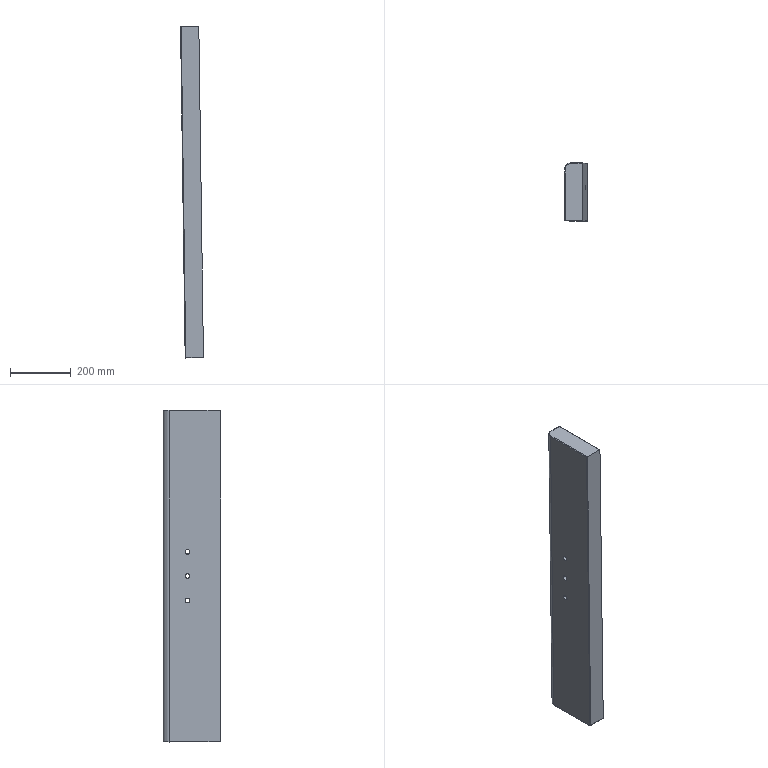Component | SolidWorks | DA-0220-Part8-5 | 1 solid | 23 faces | box 75.24 x 189.53 x 1090.68 mm | volume 12261983 mm3 | cylinder 14 | plane 6 | torus 2 | sphere 1 | commonest cylinder face diameters 4 x7 16 x6 40 x1
build123d program:
from build123d import *

# Parameters (mm, degrees)
SKETCH1_W           = 60
SKETCH1_H           = 189.5
BOSS_EXTRUDE1_DEPTH = 545
FILLET1_R           = 20
FILLET2_R           = 2
SKETCH1_2_R         = 8
CUT_EXTRUDE1_DEPTH  = 581.117


with BuildPart() as part:
    # Sketch1 → Boss-Extrude1 (new, symmetric)
    with BuildSketch(Plane.XY):
        with Locations((30, 94.75)):
            Rectangle(SKETCH1_W, SKETCH1_H)
    extrude(amount=BOSS_EXTRUDE1_DEPTH, both=True)

    # Fillet1
    fillet1_edges = [part.edges().sort_by_distance(p)[0] for p in [
        (60, 189.5, 0),
    ]]
    fillet(fillet1_edges, radius=FILLET1_R)

    # Fillet2
    fillet2_edges = [part.edges().sort_by_distance(p)[0] for p in [
        (20, 189.5, -545),
        (20, 189.5, 545),
        (54.142, 183.642, -545),
        (54.142, 183.642, 545),
        (30, 0, 545),
        (0, 94.75, -545),
        (60, 84.75, -545),
        (60, 84.75, 545),
        (60, 0, 0),
    ]]
    fillet(fillet2_edges, radius=FILLET2_R)

    # Sketch1_2 → Cut-Extrude1 (cut, through all)
    with BuildSketch(Plane(origin=(60, 0, 0), x_dir=(0, 0, -1), z_dir=(1, 0, 0))):
        with Locations(Location((80, 109.5, 0), (0, 0, 90))):
            Circle(SKETCH1_2_R)
        with Locations(Location((0, 109.5, 0), (0, 0, 90))):
            Circle(SKETCH1_2_R)
        with Locations(Location((-80, 109.5, 0), (0, 0, 90))):
            Circle(SKETCH1_2_R)
    extrude(amount=-CUT_EXTRUDE1_DEPTH, mode=Mode.SUBTRACT)


solid = part.part

# Placed as in the assembly
solid = solid.moved(Location((302.195, -203.43, 7.718), (-180, 0.7995, 179.977)))
STEP:
#1=CARTESIAN_POINT('',(11.94,-4.013,-2.845));
#2=VERTEX_POINT('',#1);
#3=CARTESIAN_POINT('',(11.94,-3.383,-2.845));
#4=VERTEX_POINT('',#3);
#5=CARTESIAN_POINT('',(11.94,-3.698,-2.845));
#6=DIRECTION('',(-0.9999,-0.000404,-0.01395));
#7=DIRECTION('',(-0.000404,1.,-0.00000282));
#8=AXIS2_PLACEMENT_3D('',#5,#6,#7);
#9=CIRCLE('',#8,0.315);
#10=EDGE_CURVE('',#2,#4,#9,.T.);
#11=ORIENTED_EDGE('',*,*,#10,.F.);
#12=CARTESIAN_POINT('',(9.578,-4.014,-2.878));
#13=VERTEX_POINT('',#12);
#14=CARTESIAN_POINT('',(11.94,-4.013,-2.845));
#15=DIRECTION('',(-0.9999,-0.000404,-0.01395));
#16=VECTOR('',#15,39.37);
#17=LINE('',#14,#16);
#18=EDGE_CURVE('',#2,#13,#17,.T.);
#19=ORIENTED_EDGE('',*,*,#18,.T.);
#20=CARTESIAN_POINT('',(9.578,-3.384,-2.878));
#21=VERTEX_POINT('',#20);
#22=CARTESIAN_POINT('',(9.578,-3.699,-2.878));
#23=DIRECTION('',(-0.9999,-0.000404,-0.01395));
#24=DIRECTION('',(-0.000404,1.,-0.00000282));
#25=AXIS2_PLACEMENT_3D('',#22,#23,#24);
#26=CIRCLE('',#25,0.315);
#27=EDGE_CURVE('',#13,#21,#26,.T.);
#28=ORIENTED_EDGE('',*,*,#27,.T.);
#29=CARTESIAN_POINT('',(11.94,-3.383,-2.845));
#30=DIRECTION('',(-0.9999,-0.000404,-0.01395));
#31=VECTOR('',#30,39.37);
#32=LINE('',#29,#31);
#33=EDGE_CURVE('',#4,#21,#32,.T.);
#34=ORIENTED_EDGE('',*,*,#33,.F.);
#35=EDGE_LOOP('',(#11,#19,#28,#34));
#36=FACE_OUTER_BOUND('',#35,.T.);
#37=CARTESIAN_POINT('',(11.94,-3.698,-2.845));
#38=DIRECTION('',(-0.9999,-0.000404,-0.01395));
#39=DIRECTION('',(-0.000404,1.,-0.00000282));
#40=AXIS2_PLACEMENT_3D('',#37,#38,#39);
#41=CYLINDRICAL_SURFACE('',#40,0.315);
#42=ADVANCED_FACE('',(#36),#41,.F.);
#43=CARTESIAN_POINT('',(11.896,-4.013,0.3038));
#44=VERTEX_POINT('',#43);
#45=CARTESIAN_POINT('',(11.896,-3.383,0.3038));
#46=VERTEX_POINT('',#45);
#47=CARTESIAN_POINT('',(11.896,-3.698,0.3038));
#48=DIRECTION('',(-0.9999,-0.000404,-0.01395));
#49=DIRECTION('',(-0.000404,1.,-0.00000282));
#50=AXIS2_PLACEMENT_3D('',#47,#48,#49);
#51=CIRCLE('',#50,0.315);
#52=EDGE_CURVE('',#44,#46,#51,.T.);
#53=ORIENTED_EDGE('',*,*,#52,.F.);
#54=CARTESIAN_POINT('',(9.534,-4.014,0.2709));
#55=VERTEX_POINT('',#54);
#56=CARTESIAN_POINT('',(11.896,-4.013,0.3038));
#57=DIRECTION('',(-0.9999,-0.000404,-0.01395));
#58=VECTOR('',#57,39.37);
#59=LINE('',#56,#58);
#60=EDGE_CURVE('',#44,#55,#59,.T.);
#61=ORIENTED_EDGE('',*,*,#60,.T.);
#62=CARTESIAN_POINT('',(9.534,-3.384,0.2709));
#63=VERTEX_POINT('',#62);
#64=CARTESIAN_POINT('',(9.534,-3.699,0.2709));
#65=DIRECTION('',(-0.9999,-0.000404,-0.01395));
#66=DIRECTION('',(-0.000404,1.,-0.00000282));
#67=AXIS2_PLACEMENT_3D('',#64,#65,#66);
#68=CIRCLE('',#67,0.315);
#69=EDGE_CURVE('',#55,#63,#68,.T.);
#70=ORIENTED_EDGE('',*,*,#69,.T.);
#71=CARTESIAN_POINT('',(11.896,-3.383,0.3038));
#72=DIRECTION('',(-0.9999,-0.000404,-0.01395));
#73=VECTOR('',#72,39.37);
#74=LINE('',#71,#73);
#75=EDGE_CURVE('',#46,#63,#74,.T.);
#76=ORIENTED_EDGE('',*,*,#75,.F.);
#77=EDGE_LOOP('',(#53,#61,#70,#76));
#78=FACE_OUTER_BOUND('',#77,.T.);
#79=CARTESIAN_POINT('',(11.896,-3.698,0.3038));
#80=DIRECTION('',(-0.9999,-0.000404,-0.01395));
#81=DIRECTION('',(-0.000404,1.,-0.00000282));
#82=AXIS2_PLACEMENT_3D('',#79,#80,#81);
#83=CYLINDRICAL_SURFACE('',#82,0.315);
#84=ADVANCED_FACE('',(#78),#83,.F.);
#85=CARTESIAN_POINT('',(11.852,-4.013,3.453));
#86=VERTEX_POINT('',#85);
#87=CARTESIAN_POINT('',(11.852,-3.383,3.453));
#88=VERTEX_POINT('',#87);
#89=CARTESIAN_POINT('',(11.852,-3.698,3.453));
#90=DIRECTION('',(-0.9999,-0.000404,-0.01395));
#91=DIRECTION('',(-0.000404,1.,-0.00000282));
#92=AXIS2_PLACEMENT_3D('',#89,#90,#91);
#93=CIRCLE('',#92,0.315);
#94=EDGE_CURVE('',#86,#88,#93,.T.);
#95=ORIENTED_EDGE('',*,*,#94,.F.);
#96=CARTESIAN_POINT('',(9.49,-4.014,3.42));
#97=VERTEX_POINT('',#96);
#98=CARTESIAN_POINT('',(11.852,-4.013,3.453));
#99=DIRECTION('',(-0.9999,-0.000404,-0.01395));
#100=VECTOR('',#99,39.37);
#101=LINE('',#98,#100);
#102=EDGE_CURVE('',#86,#97,#101,.T.);
#103=ORIENTED_EDGE('',*,*,#102,.T.);
#104=CARTESIAN_POINT('',(9.49,-3.384,3.42));
#105=VERTEX_POINT('',#104);
#106=CARTESIAN_POINT('',(9.49,-3.699,3.42));
#107=DIRECTION('',(-0.9999,-0.000404,-0.01395));
#108=DIRECTION('',(-0.000404,1.,-0.00000282));
#109=AXIS2_PLACEMENT_3D('',#106,#107,#108);
#110=CIRCLE('',#109,0.315);
#111=EDGE_CURVE('',#97,#105,#110,.T.);
#112=ORIENTED_EDGE('',*,*,#111,.T.);
#113=CARTESIAN_POINT('',(11.852,-3.383,3.453));
#114=DIRECTION('',(-0.9999,-0.000404,-0.01395));
#115=VECTOR('',#114,39.37);
#116=LINE('',#113,#115);
#117=EDGE_CURVE('',#88,#105,#116,.T.);
#118=ORIENTED_EDGE('',*,*,#117,.F.);
#119=EDGE_LOOP('',(#95,#103,#112,#118));
#120=FACE_OUTER_BOUND('',#119,.T.);
#121=CARTESIAN_POINT('',(11.852,-3.698,3.453));
#122=DIRECTION('',(-0.9999,-0.000404,-0.01395));
#123=DIRECTION('',(-0.000404,1.,-0.00000282));
#124=AXIS2_PLACEMENT_3D('',#121,#122,#123);
#125=CYLINDRICAL_SURFACE('',#124,0.315);
#126=ADVANCED_FACE('',(#120),#125,.F.);
#127=CARTESIAN_POINT('',(12.196,-8.009,-21.072));
#128=VERTEX_POINT('',#127);
#129=CARTESIAN_POINT('',(11.599,-8.009,21.68));
#130=VERTEX_POINT('',#129);
#131=CARTESIAN_POINT('',(12.197,-8.009,-21.151));
#132=DIRECTION('',(-0.01395,-0.00000282,0.9999));
#133=VECTOR('',#132,39.37);
#134=LINE('',#131,#133);
#135=EDGE_CURVE('',#128,#130,#134,.T.);
#136=ORIENTED_EDGE('',*,*,#135,.T.);
#137=CARTESIAN_POINT('',(11.519,-8.009,21.757));
#138=VERTEX_POINT('',#137);
#139=CARTESIAN_POINT('',(11.52,-8.009,21.679));
#140=DIRECTION('',(0.000404,-1.,0.00000282));
#141=DIRECTION('',(0.9999,0.000404,0.01395));
#142=AXIS2_PLACEMENT_3D('',#139,#140,#141);
#143=CIRCLE('',#142,0.07874);
#144=EDGE_CURVE('',#130,#138,#143,.T.);
#145=ORIENTED_EDGE('',*,*,#144,.T.);
#146=CARTESIAN_POINT('',(9.315,-8.01,21.727));
#147=VERTEX_POINT('',#146);
#148=CARTESIAN_POINT('',(9.236,-8.01,21.725));
#149=DIRECTION('',(-0.9999,-0.000404,-0.01395));
#150=VECTOR('',#149,39.37);
#151=LINE('',#148,#150);
#152=EDGE_CURVE('',#138,#147,#151,.T.);
#153=ORIENTED_EDGE('',*,*,#152,.T.);
#154=CARTESIAN_POINT('',(9.912,-8.01,-21.104));
#155=VERTEX_POINT('',#154);
#156=CARTESIAN_POINT('',(9.914,-8.01,-21.183));
#157=DIRECTION('',(0.01395,0.00000282,-0.9999));
#158=VECTOR('',#157,39.37);
#159=LINE('',#156,#158);
#160=EDGE_CURVE('',#147,#155,#159,.T.);
#161=ORIENTED_EDGE('',*,*,#160,.T.);
#162=CARTESIAN_POINT('',(9.834,-8.01,-21.105));
#163=DIRECTION('',(0.9999,0.000404,0.01395));
#164=VECTOR('',#163,39.37);
#165=LINE('',#162,#164);
#166=EDGE_CURVE('',#155,#128,#165,.T.);
#167=ORIENTED_EDGE('',*,*,#166,.T.);
#168=EDGE_LOOP('',(#136,#145,#153,#161,#167));
#169=FACE_OUTER_BOUND('',#168,.T.);
#170=CARTESIAN_POINT('',(9.835,-8.01,-21.184));
#171=DIRECTION('',(-0.000404,1.,-0.00000282));
#172=DIRECTION('',(0.9999,0.000404,0.01395));
#173=AXIS2_PLACEMENT_3D('',#170,#171,#172);
#174=PLANE('',#173);
#175=ADVANCED_FACE('',(#169),#174,.F.);
#176=CARTESIAN_POINT('',(9.578,-3.699,-2.878));
#177=DIRECTION('',(-0.9999,-0.000404,-0.01395));
#178=DIRECTION('',(-0.000404,1.,-0.00000282));
#179=AXIS2_PLACEMENT_3D('',#176,#177,#178);
#180=CIRCLE('',#179,0.315);
#181=EDGE_CURVE('',#21,#13,#180,.T.);
#182=ORIENTED_EDGE('',*,*,#181,.F.);
#183=ORIENTED_EDGE('',*,*,#27,.F.);
#184=EDGE_LOOP('',(#182,#183));
#185=FACE_BOUND('',#184,.T.);
#186=CARTESIAN_POINT('',(9.534,-3.699,0.2709));
#187=DIRECTION('',(-0.9999,-0.000404,-0.01395));
#188=DIRECTION('',(-0.000404,1.,-0.00000282));
#189=AXIS2_PLACEMENT_3D('',#186,#187,#188);
#190=CIRCLE('',#189,0.315);
#191=EDGE_CURVE('',#63,#55,#190,.T.);
#192=ORIENTED_EDGE('',*,*,#191,.F.);
#193=ORIENTED_EDGE('',*,*,#69,.F.);
#194=EDGE_LOOP('',(#192,#193));
#195=FACE_BOUND('',#194,.T.);
#196=CARTESIAN_POINT('',(9.49,-3.699,3.42));
#197=DIRECTION('',(-0.9999,-0.000404,-0.01395));
#198=DIRECTION('',(-0.000404,1.,-0.00000282));
#199=AXIS2_PLACEMENT_3D('',#196,#197,#198);
#200=CIRCLE('',#199,0.315);
#201=EDGE_CURVE('',#105,#97,#200,.T.);
#202=ORIENTED_EDGE('',*,*,#201,.F.);
#203=ORIENTED_EDGE('',*,*,#111,.F.);
#204=EDGE_LOOP('',(#202,#203));
#205=FACE_BOUND('',#204,.T.);
#206=CARTESIAN_POINT('',(9.834,-7.931,-21.105));
#207=VERTEX_POINT('',#206);
#208=CARTESIAN_POINT('',(9.237,-7.931,21.647));
#209=VERTEX_POINT('',#208);
#210=CARTESIAN_POINT('',(9.835,-7.931,-21.184));
#211=DIRECTION('',(-0.01395,-0.00000282,0.9999));
#212=VECTOR('',#211,39.37);
#213=LINE('',#210,#212);
#214=EDGE_CURVE('',#207,#209,#213,.T.);
#215=ORIENTED_EDGE('',*,*,#214,.T.);
#216=CARTESIAN_POINT('',(9.234,-1.337,21.647));
#217=VERTEX_POINT('',#216);
#218=CARTESIAN_POINT('',(9.234,-1.337,21.647));
#219=DIRECTION('',(-0.000404,1.,-0.00000282));
#220=VECTOR('',#219,39.37);
#221=LINE('',#218,#220);
#222=EDGE_CURVE('',#209,#217,#221,.T.);
#223=ORIENTED_EDGE('',*,*,#222,.T.);
#224=CARTESIAN_POINT('',(9.831,-1.337,-21.105));
#225=VERTEX_POINT('',#224);
#226=CARTESIAN_POINT('',(9.832,-1.337,-21.184));
#227=DIRECTION('',(0.01395,0.00000282,-0.9999));
#228=VECTOR('',#227,39.37);
#229=LINE('',#226,#228);
#230=EDGE_CURVE('',#217,#225,#229,.T.);
#231=ORIENTED_EDGE('',*,*,#230,.T.);
#232=CARTESIAN_POINT('',(9.831,-0.5493,-21.105));
#233=DIRECTION('',(0.000404,-1.,0.00000282));
#234=VECTOR('',#233,39.37);
#235=LINE('',#232,#234);
#236=EDGE_CURVE('',#225,#207,#235,.T.);
#237=ORIENTED_EDGE('',*,*,#236,.T.);
#238=EDGE_LOOP('',(#215,#223,#231,#237));
#239=FACE_OUTER_BOUND('',#238,.T.);
#240=CARTESIAN_POINT('',(9.832,-0.5493,-21.184));
#241=DIRECTION('',(0.9999,0.000404,0.01395));
#242=DIRECTION('',(0.000404,-1.,0.00000282));
#243=AXIS2_PLACEMENT_3D('',#240,#241,#242);
#244=PLANE('',#243);
#245=ADVANCED_FACE('',(#185,#195,#205,#239),#244,.F.);
#246=CARTESIAN_POINT('',(10.618,-0.549,-21.094));
#247=VERTEX_POINT('',#246);
#248=CARTESIAN_POINT('',(10.021,-0.5491,21.658));
#249=VERTEX_POINT('',#248);
#250=CARTESIAN_POINT('',(10.619,-0.549,-21.173));
#251=DIRECTION('',(-0.01395,-0.00000282,0.9999));
#252=VECTOR('',#251,39.37);
#253=LINE('',#250,#252);
#254=EDGE_CURVE('',#247,#249,#253,.T.);
#255=ORIENTED_EDGE('',*,*,#254,.T.);
#256=CARTESIAN_POINT('',(11.596,-0.5485,21.68));
#257=VERTEX_POINT('',#256);
#258=CARTESIAN_POINT('',(11.596,-0.5485,21.68));
#259=DIRECTION('',(0.9999,0.000404,0.01395));
#260=VECTOR('',#259,39.37);
#261=LINE('',#258,#260);
#262=EDGE_CURVE('',#249,#257,#261,.T.);
#263=ORIENTED_EDGE('',*,*,#262,.T.);
#264=CARTESIAN_POINT('',(12.193,-0.5484,-21.072));
#265=VERTEX_POINT('',#264);
#266=CARTESIAN_POINT('',(12.194,-0.5484,-21.151));
#267=DIRECTION('',(-0.01395,-0.00000282,0.9999));
#268=VECTOR('',#267,39.37);
#269=LINE('',#266,#268);
#270=EDGE_CURVE('',#265,#257,#269,.T.);
#271=ORIENTED_EDGE('',*,*,#270,.F.);
#272=CARTESIAN_POINT('',(12.193,-0.5484,-21.072));
#273=DIRECTION('',(-0.9999,-0.000404,-0.01395));
#274=VECTOR('',#273,39.37);
#275=LINE('',#272,#274);
#276=EDGE_CURVE('',#265,#247,#275,.T.);
#277=ORIENTED_EDGE('',*,*,#276,.T.);
#278=EDGE_LOOP('',(#255,#263,#271,#277));
#279=FACE_OUTER_BOUND('',#278,.T.);
#280=CARTESIAN_POINT('',(12.194,-0.5484,-21.151));
#281=DIRECTION('',(0.000404,-1.,0.00000282));
#282=DIRECTION('',(-0.01395,-0.00000282,0.9999));
#283=AXIS2_PLACEMENT_3D('',#280,#281,#282);
#284=PLANE('',#283);
#285=ADVANCED_FACE('',(#279),#284,.F.);
#286=CARTESIAN_POINT('',(11.94,-3.698,-2.845));
#287=DIRECTION('',(-0.9999,-0.000404,-0.01395));
#288=DIRECTION('',(-0.000404,1.,-0.00000282));
#289=AXIS2_PLACEMENT_3D('',#286,#287,#288);
#290=CIRCLE('',#289,0.315);
#291=EDGE_CURVE('',#4,#2,#290,.T.);
#292=ORIENTED_EDGE('',*,*,#291,.T.);
#293=ORIENTED_EDGE('',*,*,#10,.T.);
#294=EDGE_LOOP('',(#292,#293));
#295=FACE_BOUND('',#294,.T.);
#296=CARTESIAN_POINT('',(11.896,-3.698,0.3038));
#297=DIRECTION('',(-0.9999,-0.000404,-0.01395));
#298=DIRECTION('',(-0.000404,1.,-0.00000282));
#299=AXIS2_PLACEMENT_3D('',#296,#297,#298);
#300=CIRCLE('',#299,0.315);
#301=EDGE_CURVE('',#46,#44,#300,.T.);
#302=ORIENTED_EDGE('',*,*,#301,.T.);
#303=ORIENTED_EDGE('',*,*,#52,.T.);
#304=EDGE_LOOP('',(#302,#303));
#305=FACE_BOUND('',#304,.T.);
#306=CARTESIAN_POINT('',(11.852,-3.698,3.453));
#307=DIRECTION('',(-0.9999,-0.000404,-0.01395));
#308=DIRECTION('',(-0.000404,1.,-0.00000282));
#309=AXIS2_PLACEMENT_3D('',#306,#307,#308);
#310=CIRCLE('',#309,0.315);
#311=EDGE_CURVE('',#88,#86,#310,.T.);
#312=ORIENTED_EDGE('',*,*,#311,.T.);
#313=ORIENTED_EDGE('',*,*,#94,.T.);
#314=EDGE_LOOP('',(#312,#313));
#315=FACE_BOUND('',#314,.T.);
#316=CARTESIAN_POINT('',(12.194,-0.6271,-21.151));
#317=VERTEX_POINT('',#316);
#318=CARTESIAN_POINT('',(12.197,-7.93,-21.151));
#319=VERTEX_POINT('',#318);
#320=CARTESIAN_POINT('',(12.197,-8.009,-21.151));
#321=DIRECTION('',(0.000404,-1.,0.00000282));
#322=VECTOR('',#321,39.37);
#323=LINE('',#320,#322);
#324=EDGE_CURVE('',#317,#319,#323,.T.);
#325=ORIENTED_EDGE('',*,*,#324,.F.);
#326=CARTESIAN_POINT('',(12.193,-0.6271,-21.072));
#327=DIRECTION('',(0.9999,0.000404,0.01395));
#328=DIRECTION('',(-0.000404,1.,-0.00000282));
#329=AXIS2_PLACEMENT_3D('',#326,#327,#328);
#330=CIRCLE('',#329,0.07874);
#331=EDGE_CURVE('',#317,#265,#330,.T.);
#332=ORIENTED_EDGE('',*,*,#331,.T.);
#333=ORIENTED_EDGE('',*,*,#270,.T.);
#334=CARTESIAN_POINT('',(11.599,-8.009,21.68));
#335=DIRECTION('',(0.000404,-1.,0.00000282));
#336=VECTOR('',#335,39.37);
#337=LINE('',#334,#336);
#338=EDGE_CURVE('',#257,#130,#337,.T.);
#339=ORIENTED_EDGE('',*,*,#338,.T.);
#340=ORIENTED_EDGE('',*,*,#135,.F.);
#341=CARTESIAN_POINT('',(12.196,-7.93,-21.072));
#342=DIRECTION('',(0.9999,0.000404,0.01395));
#343=DIRECTION('',(-0.000404,1.,-0.00000282));
#344=AXIS2_PLACEMENT_3D('',#341,#342,#343);
#345=CIRCLE('',#344,0.07874);
#346=EDGE_CURVE('',#128,#319,#345,.T.);
#347=ORIENTED_EDGE('',*,*,#346,.T.);
#348=EDGE_LOOP('',(#325,#332,#333,#339,#340,#347));
#349=FACE_OUTER_BOUND('',#348,.T.);
#350=CARTESIAN_POINT('',(12.197,-8.009,-21.151));
#351=DIRECTION('',(-0.9999,-0.000404,-0.01395));
#352=DIRECTION('',(-0.000404,1.,-0.00000282));
#353=AXIS2_PLACEMENT_3D('',#350,#351,#352);
#354=PLANE('',#353);
#355=ADVANCED_FACE('',(#295,#305,#315,#349),#354,.F.);
#356=CARTESIAN_POINT('',(9.911,-1.337,-21.183));
#357=VERTEX_POINT('',#356);
#358=CARTESIAN_POINT('',(10.619,-0.6278,-21.173));
#359=VERTEX_POINT('',#358);
#360=CARTESIAN_POINT('',(10.619,-1.336,-21.173));
#361=DIRECTION('',(0.01395,0.00000282,-0.9999));
#362=DIRECTION('',(0.9999,0.000404,0.01395));
#363=AXIS2_PLACEMENT_3D('',#360,#361,#362);
#364=CIRCLE('',#363,0.7087);
#365=EDGE_CURVE('',#357,#359,#364,.T.);
#366=ORIENTED_EDGE('',*,*,#365,.T.);
#367=CARTESIAN_POINT('',(12.194,-0.6271,-21.151));
#368=DIRECTION('',(0.9999,0.000404,0.01395));
#369=VECTOR('',#368,39.37);
#370=LINE('',#367,#369);
#371=EDGE_CURVE('',#359,#317,#370,.T.);
#372=ORIENTED_EDGE('',*,*,#371,.T.);
#373=ORIENTED_EDGE('',*,*,#324,.T.);
#374=CARTESIAN_POINT('',(9.914,-7.931,-21.183));
#375=VERTEX_POINT('',#374);
#376=CARTESIAN_POINT('',(12.197,-7.93,-21.151));
#377=DIRECTION('',(-0.9999,-0.000404,-0.01395));
#378=VECTOR('',#377,39.37);
#379=LINE('',#376,#378);
#380=EDGE_CURVE('',#319,#375,#379,.T.);
#381=ORIENTED_EDGE('',*,*,#380,.T.);
#382=CARTESIAN_POINT('',(9.914,-8.01,-21.183));
#383=DIRECTION('',(-0.000404,1.,-0.00000282));
#384=VECTOR('',#383,39.37);
#385=LINE('',#382,#384);
#386=EDGE_CURVE('',#375,#357,#385,.T.);
#387=ORIENTED_EDGE('',*,*,#386,.T.);
#388=EDGE_LOOP('',(#366,#372,#373,#381,#387));
#389=FACE_OUTER_BOUND('',#388,.T.);
#390=CARTESIAN_POINT('',(12.197,-8.009,-21.151));
#391=DIRECTION('',(-0.01395,-0.00000282,0.9999));
#392=DIRECTION('',(0.9999,0.000404,0.01395));
#393=AXIS2_PLACEMENT_3D('',#390,#391,#392);
#394=PLANE('',#393);
#395=ADVANCED_FACE('',(#389),#394,.F.);
#396=ORIENTED_EDGE('',*,*,#152,.F.);
#397=CARTESIAN_POINT('',(11.516,-0.6273,21.757));
#398=VERTEX_POINT('',#397);
#399=CARTESIAN_POINT('',(11.516,-0.5485,21.757));
#400=DIRECTION('',(-0.000404,1.,-0.00000282));
#401=VECTOR('',#400,39.37);
#402=LINE('',#399,#401);
#403=EDGE_CURVE('',#138,#398,#402,.T.);
#404=ORIENTED_EDGE('',*,*,#403,.T.);
#405=CARTESIAN_POINT('',(10.02,-0.6279,21.736));
#406=VERTEX_POINT('',#405);
#407=CARTESIAN_POINT('',(10.02,-0.6279,21.736));
#408=DIRECTION('',(-0.9999,-0.000404,-0.01395));
#409=VECTOR('',#408,39.37);
#410=LINE('',#407,#409);
#411=EDGE_CURVE('',#398,#406,#410,.T.);
#412=ORIENTED_EDGE('',*,*,#411,.T.);
#413=CARTESIAN_POINT('',(9.312,-1.337,21.727));
#414=VERTEX_POINT('',#413);
#415=CARTESIAN_POINT('',(10.021,-1.337,21.736));
#416=DIRECTION('',(-0.01395,-0.00000282,0.9999));
#417=DIRECTION('',(0.9999,0.000404,0.01395));
#418=AXIS2_PLACEMENT_3D('',#415,#416,#417);
#419=CIRCLE('',#418,0.7087);
#420=EDGE_CURVE('',#406,#414,#419,.T.);
#421=ORIENTED_EDGE('',*,*,#420,.T.);
#422=CARTESIAN_POINT('',(9.315,-8.01,21.727));
#423=DIRECTION('',(0.000404,-1.,0.00000282));
#424=VECTOR('',#423,39.37);
#425=LINE('',#422,#424);
#426=EDGE_CURVE('',#414,#147,#425,.T.);
#427=ORIENTED_EDGE('',*,*,#426,.T.);
#428=EDGE_LOOP('',(#396,#404,#412,#421,#427));
#429=FACE_OUTER_BOUND('',#428,.T.);
#430=CARTESIAN_POINT('',(11.598,-8.009,21.758));
#431=DIRECTION('',(-0.01395,-0.00000282,0.9999));
#432=DIRECTION('',(0.9999,0.000404,0.01395));
#433=AXIS2_PLACEMENT_3D('',#430,#431,#432);
#434=PLANE('',#433);
#435=ADVANCED_FACE('',(#429),#434,.T.);
#436=ORIENTED_EDGE('',*,*,#230,.F.);
#437=CARTESIAN_POINT('',(10.022,-1.337,21.658));
#438=DIRECTION('',(0.01395,0.00000282,-0.9999));
#439=DIRECTION('',(0.9999,0.000404,0.01395));
#440=AXIS2_PLACEMENT_3D('',#437,#438,#439);
#441=CIRCLE('',#440,0.7874);
#442=EDGE_CURVE('',#217,#249,#441,.T.);
#443=ORIENTED_EDGE('',*,*,#442,.T.);
#444=ORIENTED_EDGE('',*,*,#254,.F.);
#445=CARTESIAN_POINT('',(10.618,-1.336,-21.094));
#446=DIRECTION('',(-0.01395,-0.00000282,0.9999));
#447=DIRECTION('',(0.9999,0.000404,0.01395));
#448=AXIS2_PLACEMENT_3D('',#445,#446,#447);
#449=CIRCLE('',#448,0.7874);
#450=EDGE_CURVE('',#247,#225,#449,.T.);
#451=ORIENTED_EDGE('',*,*,#450,.T.);
#452=EDGE_LOOP('',(#436,#443,#444,#451));
#453=FACE_OUTER_BOUND('',#452,.T.);
#454=CARTESIAN_POINT('',(10.619,-1.336,-21.173));
#455=DIRECTION('',(-0.01395,-0.00000282,0.9999));
#456=DIRECTION('',(0.9999,0.000404,0.01395));
#457=AXIS2_PLACEMENT_3D('',#454,#455,#456);
#458=CYLINDRICAL_SURFACE('',#457,0.7874);
#459=ADVANCED_FACE('',(#453),#458,.T.);
#460=ORIENTED_EDGE('',*,*,#331,.F.);
#461=ORIENTED_EDGE('',*,*,#371,.F.);
#462=CARTESIAN_POINT('',(10.618,-0.6278,-21.094));
#463=DIRECTION('',(-0.9999,-0.000404,-0.01395));
#464=DIRECTION('',(-0.01395,-0.00000282,0.9999));
#465=AXIS2_PLACEMENT_3D('',#462,#463,#464);
#466=CIRCLE('',#465,0.07874);
#467=EDGE_CURVE('',#247,#359,#466,.T.);
#468=ORIENTED_EDGE('',*,*,#467,.F.);
#469=ORIENTED_EDGE('',*,*,#276,.F.);
#470=EDGE_LOOP('',(#460,#461,#468,#469));
#471=FACE_OUTER_BOUND('',#470,.T.);
#472=CARTESIAN_POINT('',(12.193,-0.6271,-21.072));
#473=DIRECTION('',(0.9999,0.000404,0.01395));
#474=DIRECTION('',(0.01395,0.00000282,-0.9999));
#475=AXIS2_PLACEMENT_3D('',#472,#473,#474);
#476=CYLINDRICAL_SURFACE('',#475,0.07874);
#477=ADVANCED_FACE('',(#471),#476,.T.);
#478=ORIENTED_EDGE('',*,*,#467,.T.);
#479=ORIENTED_EDGE('',*,*,#365,.F.);
#480=CARTESIAN_POINT('',(9.91,-1.337,-21.104));
#481=DIRECTION('',(0.000404,-1.,0.00000282));
#482=DIRECTION('',(-0.01395,-0.00000282,0.9999));
#483=AXIS2_PLACEMENT_3D('',#480,#481,#482);
#484=CIRCLE('',#483,0.07874);
#485=EDGE_CURVE('',#225,#357,#484,.T.);
#486=ORIENTED_EDGE('',*,*,#485,.F.);
#487=ORIENTED_EDGE('',*,*,#450,.F.);
#488=EDGE_LOOP('',(#478,#479,#486,#487));
#489=FACE_OUTER_BOUND('',#488,.T.);
#490=CARTESIAN_POINT('',(10.618,-1.336,-21.094));
#491=DIRECTION('',(-0.01395,-0.00000282,0.9999));
#492=DIRECTION('',(0.9999,0.000404,0.01395));
#493=AXIS2_PLACEMENT_3D('',#490,#491,#492);
#494=TOROIDAL_SURFACE('',#493,0.7087,0.07874);
#495=ADVANCED_FACE('',(#489),#494,.T.);
#496=ORIENTED_EDGE('',*,*,#346,.F.);
#497=ORIENTED_EDGE('',*,*,#166,.F.);
#498=CARTESIAN_POINT('',(9.912,-7.931,-21.104));
#499=DIRECTION('',(-0.9999,-0.000404,-0.01395));
#500=DIRECTION('',(-0.01395,-0.00000282,0.9999));
#501=AXIS2_PLACEMENT_3D('',#498,#499,#500);
#502=CIRCLE('',#501,0.07874);
#503=EDGE_CURVE('',#375,#155,#502,.T.);
#504=ORIENTED_EDGE('',*,*,#503,.F.);
#505=ORIENTED_EDGE('',*,*,#380,.F.);
#506=EDGE_LOOP('',(#496,#497,#504,#505));
#507=FACE_OUTER_BOUND('',#506,.T.);
#508=CARTESIAN_POINT('',(12.196,-7.93,-21.072));
#509=DIRECTION('',(-0.9999,-0.000404,-0.01395));
#510=DIRECTION('',(-0.000404,1.,-0.00000282));
#511=AXIS2_PLACEMENT_3D('',#508,#509,#510);
#512=CYLINDRICAL_SURFACE('',#511,0.07874);
#513=ADVANCED_FACE('',(#507),#512,.T.);
#514=ORIENTED_EDGE('',*,*,#485,.T.);
#515=ORIENTED_EDGE('',*,*,#386,.F.);
#516=CARTESIAN_POINT('',(9.912,-7.931,-21.104));
#517=DIRECTION('',(0.000404,-1.,0.00000282));
#518=DIRECTION('',(-0.01395,-0.00000282,0.9999));
#519=AXIS2_PLACEMENT_3D('',#516,#517,#518);
#520=CIRCLE('',#519,0.07874);
#521=EDGE_CURVE('',#207,#375,#520,.T.);
#522=ORIENTED_EDGE('',*,*,#521,.F.);
#523=ORIENTED_EDGE('',*,*,#236,.F.);
#524=EDGE_LOOP('',(#514,#515,#522,#523));
#525=FACE_OUTER_BOUND('',#524,.T.);
#526=CARTESIAN_POINT('',(9.912,-8.01,-21.104));
#527=DIRECTION('',(-0.000404,1.,-0.00000282));
#528=DIRECTION('',(0.9999,0.000404,0.01395));
#529=AXIS2_PLACEMENT_3D('',#526,#527,#528);
#530=CYLINDRICAL_SURFACE('',#529,0.07874);
#531=ADVANCED_FACE('',(#525),#530,.T.);
#532=ORIENTED_EDGE('',*,*,#521,.T.);
#533=ORIENTED_EDGE('',*,*,#503,.T.);
#534=CARTESIAN_POINT('',(9.912,-7.931,-21.104));
#535=DIRECTION('',(-0.01395,-0.00000282,0.9999));
#536=DIRECTION('',(-0.9999,-0.000404,-0.01395));
#537=AXIS2_PLACEMENT_3D('',#534,#535,#536);
#538=CIRCLE('',#537,0.07874);
#539=EDGE_CURVE('',#207,#155,#538,.T.);
#540=ORIENTED_EDGE('',*,*,#539,.F.);
#541=EDGE_LOOP('',(#532,#533,#540));
#542=FACE_OUTER_BOUND('',#541,.T.);
#543=CARTESIAN_POINT('',(9.912,-7.931,-21.104));
#544=DIRECTION('',(-0.000404,1.,-0.00000282));
#545=DIRECTION('',(-0.9999,-0.000404,-0.01395));
#546=AXIS2_PLACEMENT_3D('',#543,#544,#545);
#547=SPHERICAL_SURFACE('',#546,0.07874);
#548=ADVANCED_FACE('',(#542),#547,.T.);
#549=ORIENTED_EDGE('',*,*,#539,.T.);
#550=ORIENTED_EDGE('',*,*,#160,.F.);
#551=CARTESIAN_POINT('',(9.237,-7.931,21.647));
#552=CARTESIAN_POINT('',(9.236,-7.977,21.693));
#553=CARTESIAN_POINT('',(9.269,-8.01,21.726));
#554=CARTESIAN_POINT('',(9.315,-8.01,21.727));
#555=(BOUNDED_CURVE()B_SPLINE_CURVE(3,(#551,#552,#553,#554),.UNSPECIFIED.,.F.,.F.)B_SPLINE_CURVE_WITH_KNOTS((4,4),(4.712,6.283),.UNSPECIFIED.)CURVE()GEOMETRIC_REPRESENTATION_ITEM()RATIONAL_B_SPLINE_CURVE((1.,0.8047,0.8047,1.))REPRESENTATION_ITEM(''));
#556=EDGE_CURVE('',#209,#147,#555,.T.);
#557=ORIENTED_EDGE('',*,*,#556,.F.);
#558=ORIENTED_EDGE('',*,*,#214,.F.);
#559=EDGE_LOOP('',(#549,#550,#557,#558));
#560=FACE_OUTER_BOUND('',#559,.T.);
#561=CARTESIAN_POINT('',(9.914,-7.931,-21.183));
#562=DIRECTION('',(-0.01395,-0.00000282,0.9999));
#563=DIRECTION('',(0.9999,0.000404,0.01395));
#564=AXIS2_PLACEMENT_3D('',#561,#562,#563);
#565=CYLINDRICAL_SURFACE('',#564,0.07874);
#566=ADVANCED_FACE('',(#560),#565,.T.);
#567=ORIENTED_EDGE('',*,*,#556,.T.);
#568=ORIENTED_EDGE('',*,*,#426,.F.);
#569=CARTESIAN_POINT('',(9.313,-1.337,21.648));
#570=DIRECTION('',(-0.000404,1.,-0.00000282));
#571=DIRECTION('',(0.01395,0.00000282,-0.9999));
#572=AXIS2_PLACEMENT_3D('',#569,#570,#571);
#573=CIRCLE('',#572,0.07874);
#574=EDGE_CURVE('',#217,#414,#573,.T.);
#575=ORIENTED_EDGE('',*,*,#574,.F.);
#576=ORIENTED_EDGE('',*,*,#222,.F.);
#577=EDGE_LOOP('',(#567,#568,#575,#576));
#578=FACE_OUTER_BOUND('',#577,.T.);
#579=CARTESIAN_POINT('',(9.313,-0.5494,21.648));
#580=DIRECTION('',(0.000404,-1.,0.00000282));
#581=DIRECTION('',(-0.9999,-0.000404,-0.01395));
#582=AXIS2_PLACEMENT_3D('',#579,#580,#581);
#583=CYLINDRICAL_SURFACE('',#582,0.07874);
#584=ADVANCED_FACE('',(#578),#583,.T.);
#585=ORIENTED_EDGE('',*,*,#574,.T.);
#586=ORIENTED_EDGE('',*,*,#420,.F.);
#587=CARTESIAN_POINT('',(10.021,-0.6279,21.658));
#588=DIRECTION('',(0.9999,0.000404,0.01395));
#589=DIRECTION('',(0.01395,0.00000282,-0.9999));
#590=AXIS2_PLACEMENT_3D('',#587,#588,#589);
#591=CIRCLE('',#590,0.07874);
#592=EDGE_CURVE('',#249,#406,#591,.T.);
#593=ORIENTED_EDGE('',*,*,#592,.F.);
#594=ORIENTED_EDGE('',*,*,#442,.F.);
#595=EDGE_LOOP('',(#585,#586,#593,#594));
#596=FACE_OUTER_BOUND('',#595,.T.);
#597=CARTESIAN_POINT('',(10.022,-1.337,21.658));
#598=DIRECTION('',(-0.01395,-0.00000282,0.9999));
#599=DIRECTION('',(0.9999,0.000404,0.01395));
#600=AXIS2_PLACEMENT_3D('',#597,#598,#599);
#601=TOROIDAL_SURFACE('',#600,0.7087,0.07874);
#602=ADVANCED_FACE('',(#596),#601,.T.);
#603=ORIENTED_EDGE('',*,*,#144,.F.);
#604=ORIENTED_EDGE('',*,*,#338,.F.);
#605=CARTESIAN_POINT('',(11.516,-0.6273,21.757));
#606=CARTESIAN_POINT('',(11.562,-0.5811,21.758));
#607=CARTESIAN_POINT('',(11.595,-0.5485,21.726));
#608=CARTESIAN_POINT('',(11.596,-0.5485,21.68));
#609=(BOUNDED_CURVE()B_SPLINE_CURVE(3,(#605,#606,#607,#608),.UNSPECIFIED.,.F.,.F.)B_SPLINE_CURVE_WITH_KNOTS((4,4),(4.712,6.283),.UNSPECIFIED.)CURVE()GEOMETRIC_REPRESENTATION_ITEM()RATIONAL_B_SPLINE_CURVE((1.,0.8047,0.8047,1.))REPRESENTATION_ITEM(''));
#610=EDGE_CURVE('',#398,#257,#609,.T.);
#611=ORIENTED_EDGE('',*,*,#610,.F.);
#612=ORIENTED_EDGE('',*,*,#403,.F.);
#613=EDGE_LOOP('',(#603,#604,#611,#612));
#614=FACE_OUTER_BOUND('',#613,.T.);
#615=CARTESIAN_POINT('',(11.52,-8.009,21.679));
#616=DIRECTION('',(-0.000404,1.,-0.00000282));
#617=DIRECTION('',(0.9999,0.000404,0.01395));
#618=AXIS2_PLACEMENT_3D('',#615,#616,#617);
#619=CYLINDRICAL_SURFACE('',#618,0.07874);
#620=ADVANCED_FACE('',(#614),#619,.T.);
#621=ORIENTED_EDGE('',*,*,#592,.T.);
#622=ORIENTED_EDGE('',*,*,#411,.F.);
#623=ORIENTED_EDGE('',*,*,#610,.T.);
#624=ORIENTED_EDGE('',*,*,#262,.F.);
#625=EDGE_LOOP('',(#621,#622,#623,#624));
#626=FACE_OUTER_BOUND('',#625,.T.);
#627=CARTESIAN_POINT('',(11.596,-0.6272,21.68));
#628=DIRECTION('',(-0.9999,-0.000404,-0.01395));
#629=DIRECTION('',(-0.01395,-0.00000282,0.9999));
#630=AXIS2_PLACEMENT_3D('',#627,#628,#629);
#631=CYLINDRICAL_SURFACE('',#630,0.07874);
#632=ADVANCED_FACE('',(#626),#631,.T.);
#633=ORIENTED_EDGE('',*,*,#102,.F.);
#634=ORIENTED_EDGE('',*,*,#311,.F.);
#635=ORIENTED_EDGE('',*,*,#117,.T.);
#636=ORIENTED_EDGE('',*,*,#201,.T.);
#637=EDGE_LOOP('',(#633,#634,#635,#636));
#638=FACE_OUTER_BOUND('',#637,.T.);
#639=CARTESIAN_POINT('',(11.852,-3.698,3.453));
#640=DIRECTION('',(-0.9999,-0.000404,-0.01395));
#641=DIRECTION('',(-0.000404,1.,-0.00000282));
#642=AXIS2_PLACEMENT_3D('',#639,#640,#641);
#643=CYLINDRICAL_SURFACE('',#642,0.315);
#644=ADVANCED_FACE('',(#638),#643,.F.);
#645=ORIENTED_EDGE('',*,*,#60,.F.);
#646=ORIENTED_EDGE('',*,*,#301,.F.);
#647=ORIENTED_EDGE('',*,*,#75,.T.);
#648=ORIENTED_EDGE('',*,*,#191,.T.);
#649=EDGE_LOOP('',(#645,#646,#647,#648));
#650=FACE_OUTER_BOUND('',#649,.T.);
#651=CARTESIAN_POINT('',(11.896,-3.698,0.3038));
#652=DIRECTION('',(-0.9999,-0.000404,-0.01395));
#653=DIRECTION('',(-0.000404,1.,-0.00000282));
#654=AXIS2_PLACEMENT_3D('',#651,#652,#653);
#655=CYLINDRICAL_SURFACE('',#654,0.315);
#656=ADVANCED_FACE('',(#650),#655,.F.);
#657=ORIENTED_EDGE('',*,*,#18,.F.);
#658=ORIENTED_EDGE('',*,*,#291,.F.);
#659=ORIENTED_EDGE('',*,*,#33,.T.);
#660=ORIENTED_EDGE('',*,*,#181,.T.);
#661=EDGE_LOOP('',(#657,#658,#659,#660));
#662=FACE_OUTER_BOUND('',#661,.T.);
#663=CARTESIAN_POINT('',(11.94,-3.698,-2.845));
#664=DIRECTION('',(-0.9999,-0.000404,-0.01395));
#665=DIRECTION('',(-0.000404,1.,-0.00000282));
#666=AXIS2_PLACEMENT_3D('',#663,#664,#665);
#667=CYLINDRICAL_SURFACE('',#666,0.315);
#668=ADVANCED_FACE('',(#662),#667,.F.);
#669=CLOSED_SHELL('',(#42,#84,#126,#175,#245,#285,#355,#395,#435,#459,#477,#495,#513,#531,#548,#566,#584,#602,#620,#632,#644,#656,#668));
#670=MANIFOLD_SOLID_BREP('',#669);
#671=CARTESIAN_POINT('',(0.,0.,0.));
#672=DIRECTION('',(0.,0.,1.));
#673=DIRECTION('',(1.,0.,0.));
#674=AXIS2_PLACEMENT_3D('',#671,#672,#673);
#675=(LENGTH_UNIT()NAMED_UNIT(*)SI_UNIT($,.METRE.));
#676=LENGTH_MEASURE_WITH_UNIT(LENGTH_MEASURE(0.0254),#675);
#677=DIMENSIONAL_EXPONENTS(1.,0.,0.,0.,0.,0.,0.);
#678=(CONVERSION_BASED_UNIT('',#676)LENGTH_UNIT()NAMED_UNIT(#677));
#679=UNCERTAINTY_MEASURE_WITH_UNIT(LENGTH_MEASURE(0.00001),#678,'','');
#680=(NAMED_UNIT(*)PLANE_ANGLE_UNIT()SI_UNIT($,.RADIAN.));
#681=(NAMED_UNIT(*)SI_UNIT($,.STERADIAN.)SOLID_ANGLE_UNIT());
#682=(GEOMETRIC_REPRESENTATION_CONTEXT(3)GLOBAL_UNCERTAINTY_ASSIGNED_CONTEXT((#679))GLOBAL_UNIT_ASSIGNED_CONTEXT((#678,#680,#681))REPRESENTATION_CONTEXT('',''));
#683=ADVANCED_BREP_SHAPE_REPRESENTATION('',(#670,#674),#682);
#684=COLOUR_RGB('',0.7922,0.8196,0.9333);
#685=FILL_AREA_STYLE_COLOUR('',#684);
#686=FILL_AREA_STYLE('',(#685));
#687=SURFACE_STYLE_FILL_AREA(#686);
#688=SURFACE_SIDE_STYLE('',(#687));
#689=SURFACE_STYLE_USAGE(.BOTH.,#688);
#690=PRESENTATION_STYLE_ASSIGNMENT((#689));
#691=STYLED_ITEM('',(#690),#670);
#692=(LENGTH_UNIT()NAMED_UNIT(*)SI_UNIT($,.METRE.));
#693=LENGTH_MEASURE_WITH_UNIT(LENGTH_MEASURE(0.0254),#692);
#694=DIMENSIONAL_EXPONENTS(1.,0.,0.,0.,0.,0.,0.);
#695=(CONVERSION_BASED_UNIT('',#693)LENGTH_UNIT()NAMED_UNIT(#694));
#696=UNCERTAINTY_MEASURE_WITH_UNIT(LENGTH_MEASURE(0.00001),#695,'','');
#697=(NAMED_UNIT(*)PLANE_ANGLE_UNIT()SI_UNIT($,.RADIAN.));
#698=(NAMED_UNIT(*)SI_UNIT($,.STERADIAN.)SOLID_ANGLE_UNIT());
#699=(GEOMETRIC_REPRESENTATION_CONTEXT(3)GLOBAL_UNCERTAINTY_ASSIGNED_CONTEXT((#696))GLOBAL_UNIT_ASSIGNED_CONTEXT((#695,#697,#698))REPRESENTATION_CONTEXT('',''));
#700=MECHANICAL_DESIGN_GEOMETRIC_PRESENTATION_REPRESENTATION('',(#691),#699);
#701=PRESENTATION_LAYER_ASSIGNMENT('','',(#691));